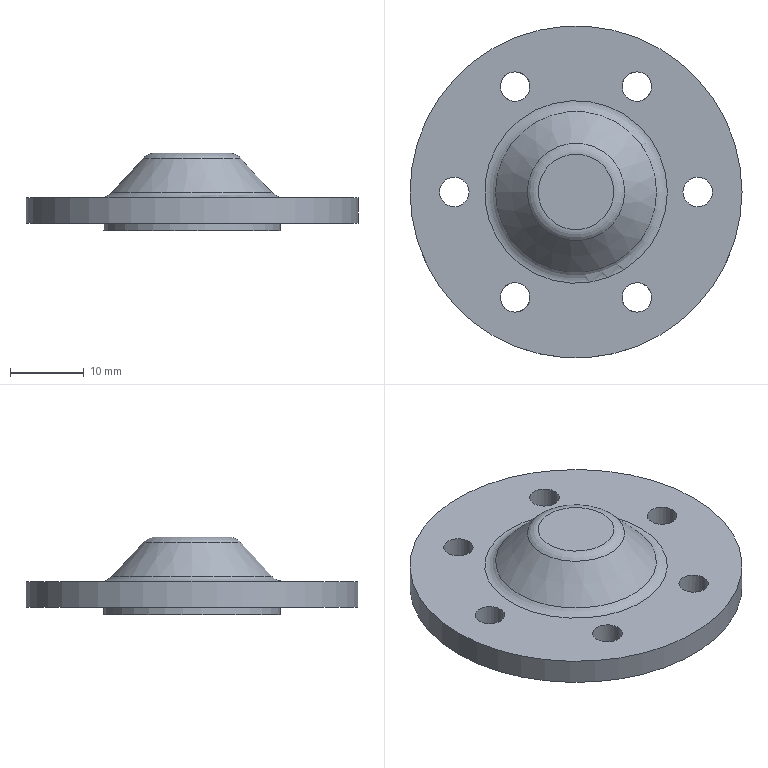Component | NX | END_CAP | 1 solid | 17 faces | volume 6571 mm3 | cylinder 9 | plane 5 | torus 2 | cone 1 | commonest cylinder face diameters 4 x6 24 x1 45 x1 12 x1